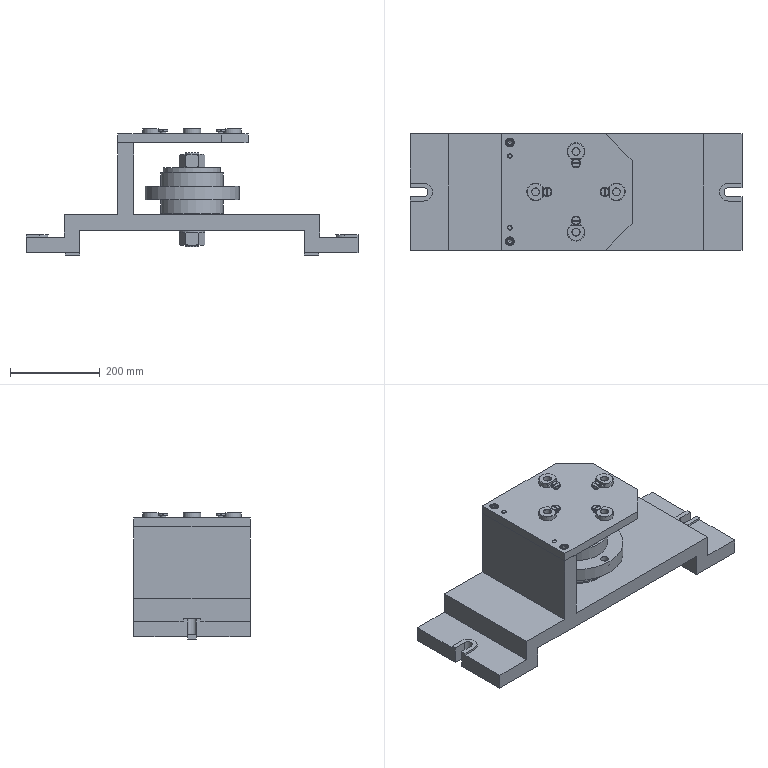Assembly | NX | mm | 24 component files | 24 solids | 418 faces | box 740 x 260 x 283 mm | volume 12577758 mm3 | plane 224 | cone 94 | cylinder 92 | torus 8 | commonest cylinder face diameters 26 x12 8 x8 20 x8 10 x8 17 x8 39 x4 30.158 x4 6 x4
Bill of materials:
unnamed part 1 | 1 |  | Flat circular disc of uniform thickness with an open-ended straight radial slot running from the outer edge to past the center, ending in a semicircular end (C-shaped / slotted washer form).
unnamed part 2 | 4 |  | Revolved pin with a large chamfered cylindrical head carrying a straight diametral slot across its top face, a short larger-diameter collar under the head, a narrow reduced-diameter neck or groove, then a plain cylindrical shank.
GB-T95-2002,M30 | 1 |  | Plain Washer, GB-T 95-2002,M30
GB-T119.1-2000,10x40 | 2 |  | Parallel Pin, GB-T 119.1-2000,10x40
unnamed part 3 | 2 |  | Rectangular block with one cylindrical hole through its center on the large face, and chamfers along the four long edges.
unnamed part 4 | 4 |  | Flanged cylindrical bushing: a larger-diameter flange on a smaller cylindrical body, with a central through bore. One side of the flange has a flat cut and a stepped notch with reduced height. The outer edges are chamfered.
GB-T70.1-2000,M6x10 | 2 |  | Hexagon Socket Head Cap Screw, GB-T 70.1-2000,M6x10
GB-T70.1-2000,M12x20 | 2 |  | Hexagon Socket Head Cap Screw, GB-T 70.1-2000,M12x20
unnamed part 5 | 1 |  | Round flange with a central hub projecting on both sides. It has a large central through bore with an internal step, and four small through holes evenly spaced on a bolt circle in the flange.
unnamed part 6 | 1 |  | Flat plate of uniform thickness, roughly rectangular with two adjacent corners chamfered on one side. It has a pattern of through holes: four larger holes in a cross arrangement, each with a smaller hole nearby toward the center, plus four holes in a column along the opposite straight edge.
GB-T41-2000,M33x3.5 | 2 |  | Hexagonal prism with a central cylindrical through-bore and chamfered edges at both ends, giving the hex-nut-like shape.
unnamed part 7 | 1 |  | Solid stepped shaft: a central large-diameter cylindrical collar with coaxial smaller-diameter journals on both sides, each stepping down again to a smaller end diameter. No visible bore.
unnamed part 8 | 1 |  | Bracket with a hat-shaped base: a raised central platform with lower end tabs, each tab having an open U-slot at its edge. A thin vertical wall stands across the platform with small holes in its top edge. The platform has a central through hole inside a shallow circular recess or boss outline.
Mates:
1. fix | fixture_body 1 component
2. concentric | flange 1 edge | fixture_body 1 edge
3. concentric | locating_pin 1 edge | flange 1 edge
4. concentric | qc_washer 1 edge | flange 1 edge
5. concentric | GB-T41-2000_M33x3_5 2 edge | qc_washer 1 edge
6. concentric | GB-T95-2002_M30 1 edge | fixture_body 1 edge
7. concentric | GB-T41-2000_M33x3_5 1 edge | GB-T95-2002_M30 1 edge
8. concentric | drill_bush 4 edge | drill_template 1 edge
9. concentric | drill_bush_screw 4 edge | drill_template 1 arc
10. touch align | drill_template 1 face | fixture_body 1 face
11. touch align | drill_bush 4 face | flange 1 face
12. bond | flange 1 component | assembly component
13. bond | drill_bush_screw 4 component | assembly component
14. bond | drill_bush 4 component | assembly component
15. bond | drill_bush_screw 3 component | assembly component
16. bond | drill_bush 3 component | assembly component
17. bond | drill_bush_screw 2 component | assembly component
18. bond | drill_bush 2 component | assembly component
19. bond | drill_bush_screw 1 component | assembly component
20. bond | drill_bush 1 component | assembly component
21. circular | assembly datumaxis | assembly cartesiancoordinatesystem | assembly cartesiancoordinatesystem | assembly cartesiancoordinatesystem | assembly cartesiancoordinatesystem
22. circular | assembly datumaxis | assembly cartesiancoordinatesystem | assembly cartesiancoordinatesystem | assembly cartesiancoordinatesystem | assembly cartesiancoordinatesystem
23. touch align | locating_key 2 face | fixture_body 1 face
24. touch align | locating_key 2 face | fixture_body 1 face
25. touch align | locating_key 2 face | fixture_body 1 face
26. bond | fixture_body 1 component | assembly component
27. bond | locating_key 2 component | assembly component
28. bond | locating_key 1 component | assembly component
29. linear | assembly datumaxis | assembly cartesiancoordinatesystem | assembly cartesiancoordinatesystem